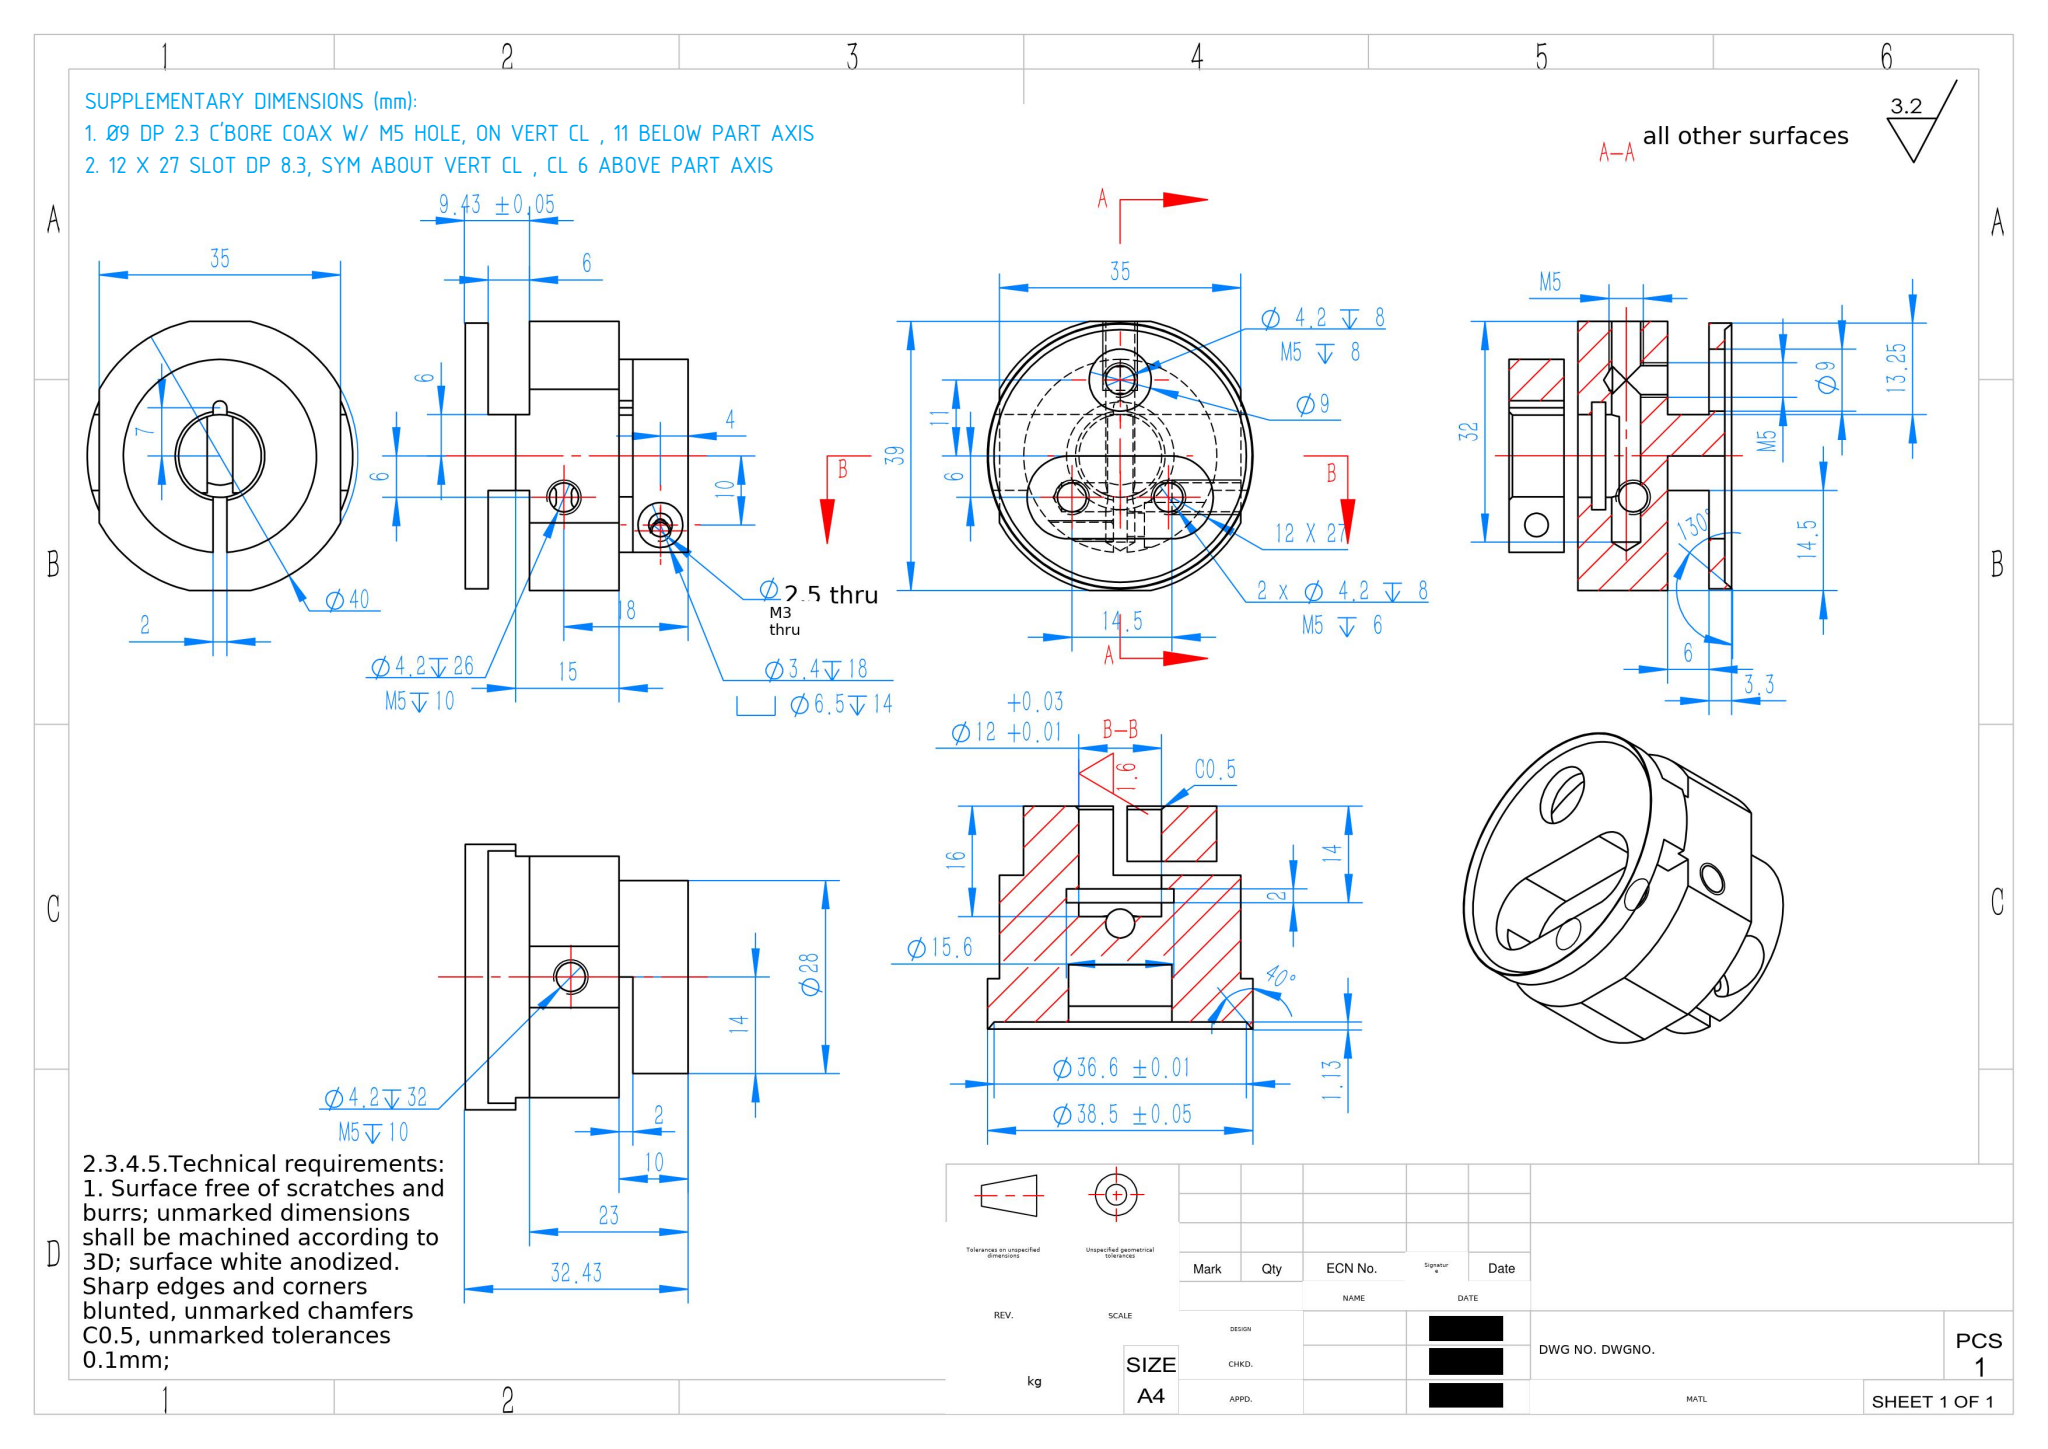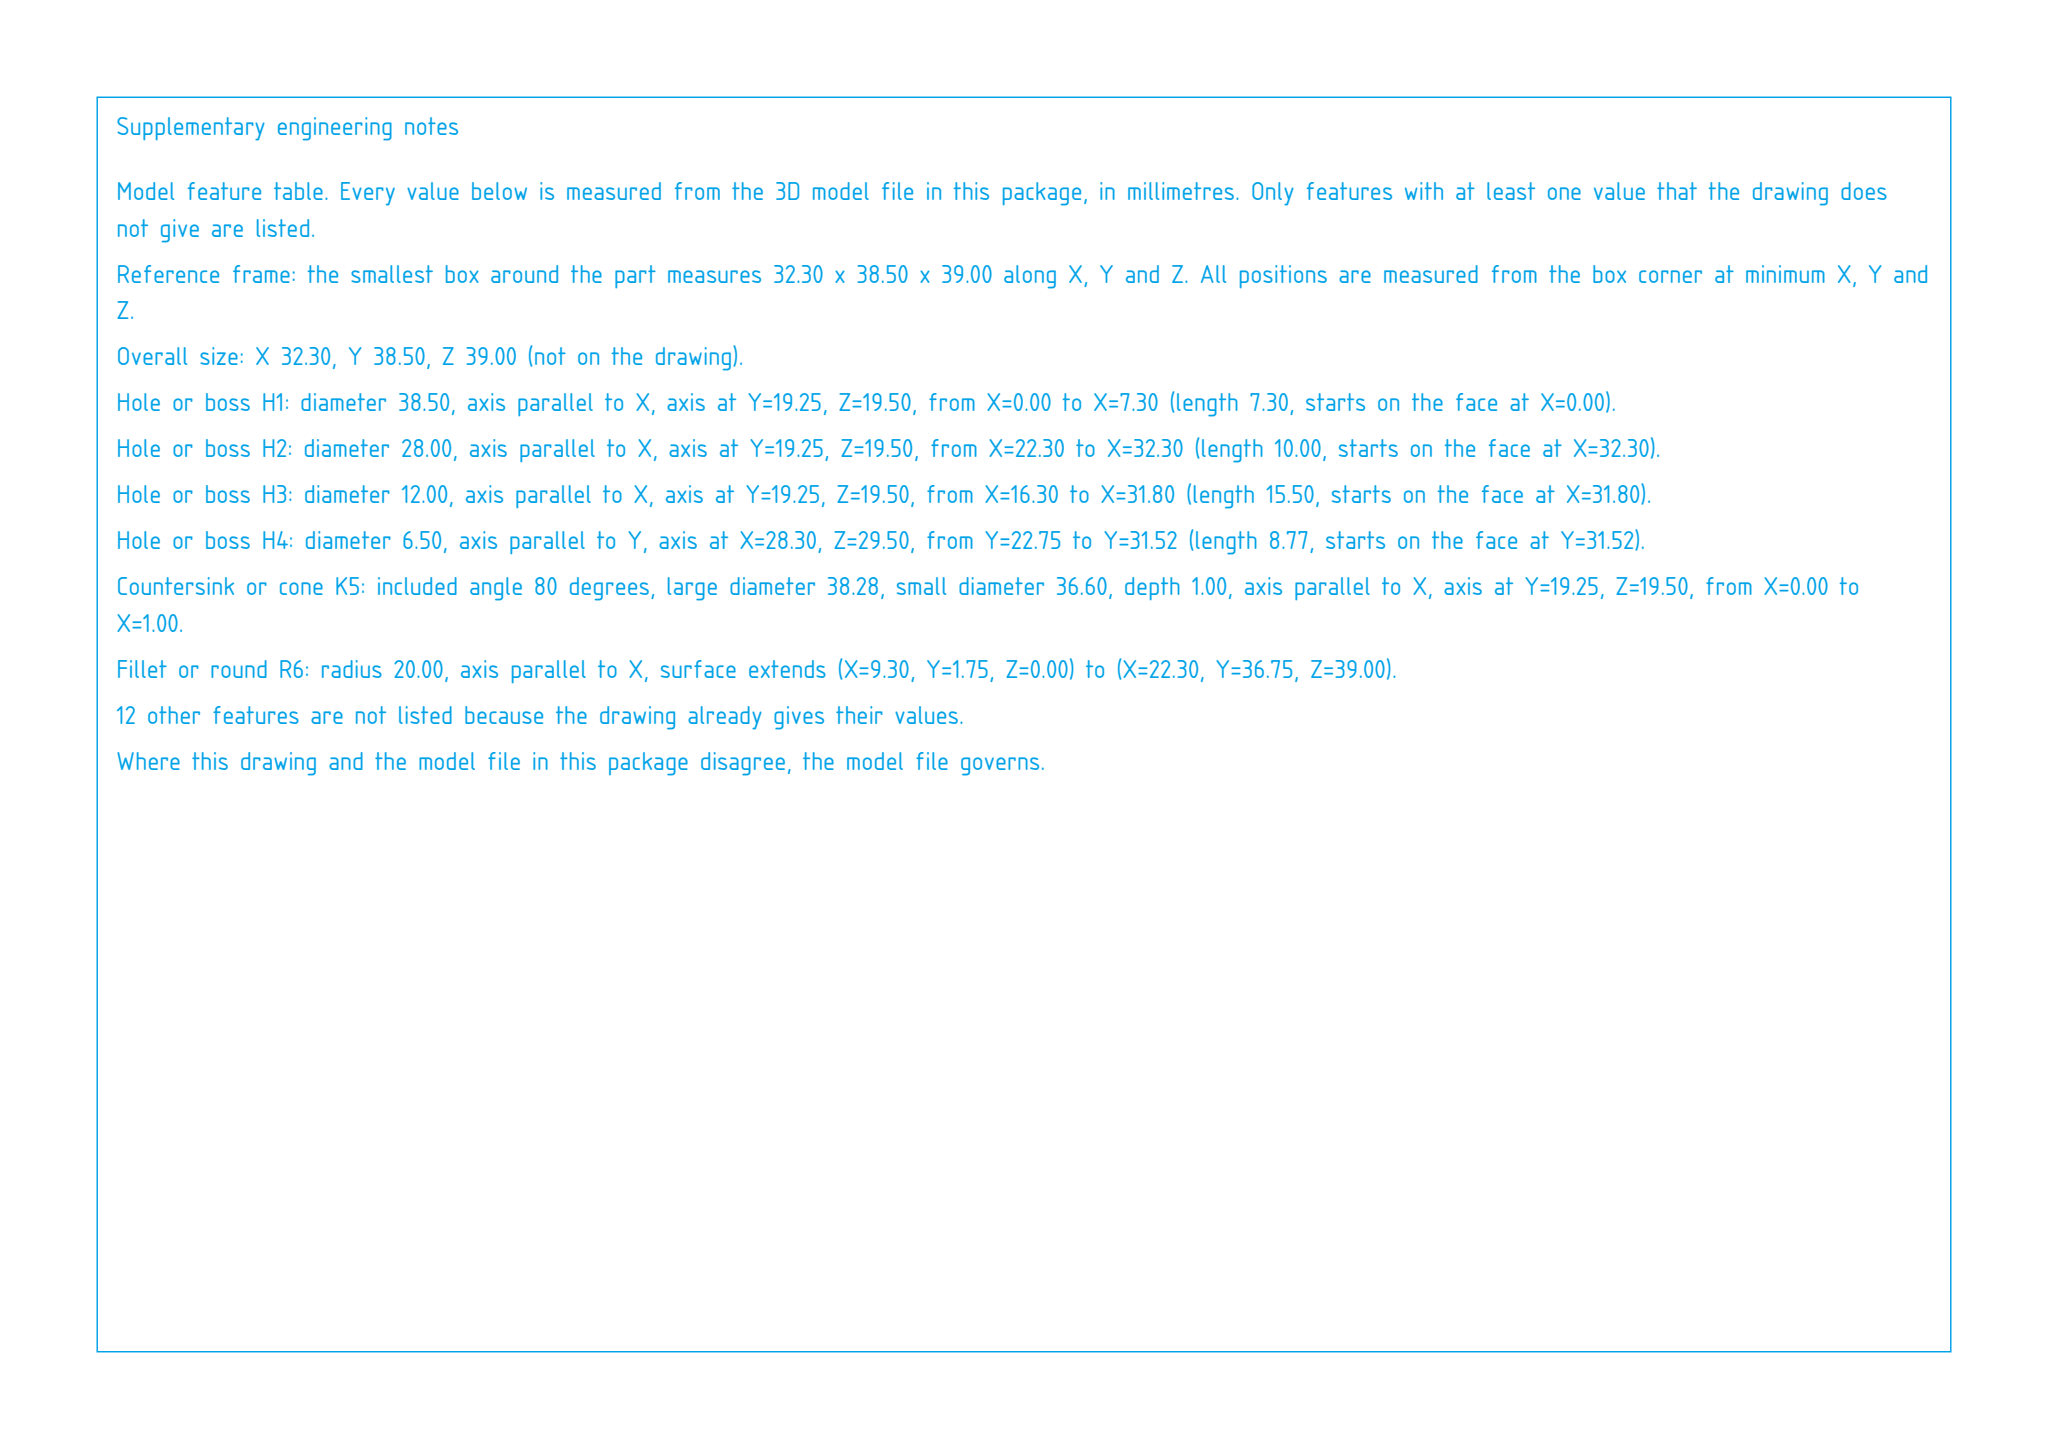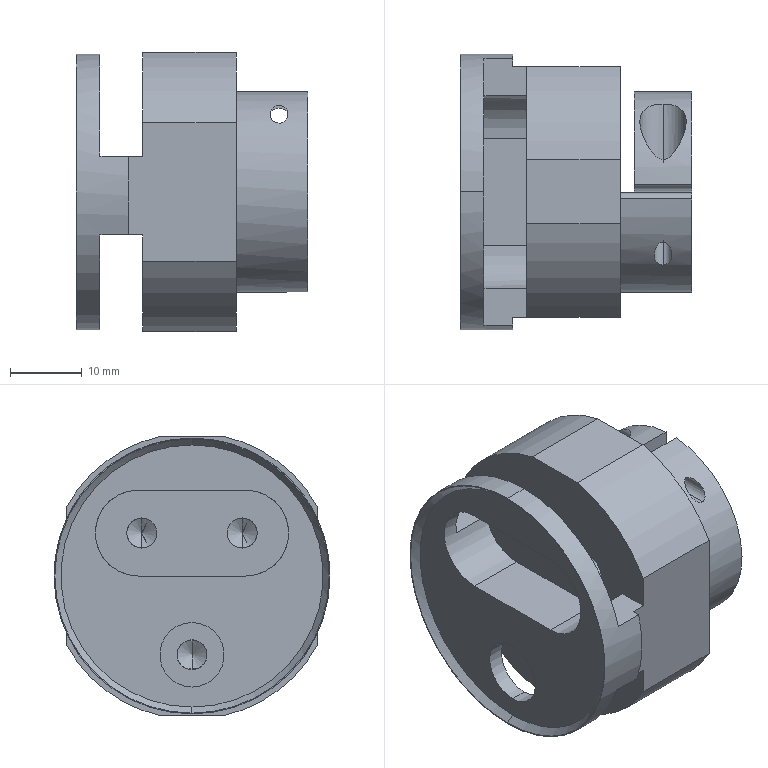Part | SolidWorks | mm | 1 solid | 97 faces | box 32.3 x 38.5 x 39 mm | volume 21356 mm3 | cylinder 52 | plane 30 | cone 15 | commonest cylinder face diameters 4.2 x26 12 x7 40 x4 15.6 x2 2.5 x2 6.5 x2 3.4 x2 2 x2